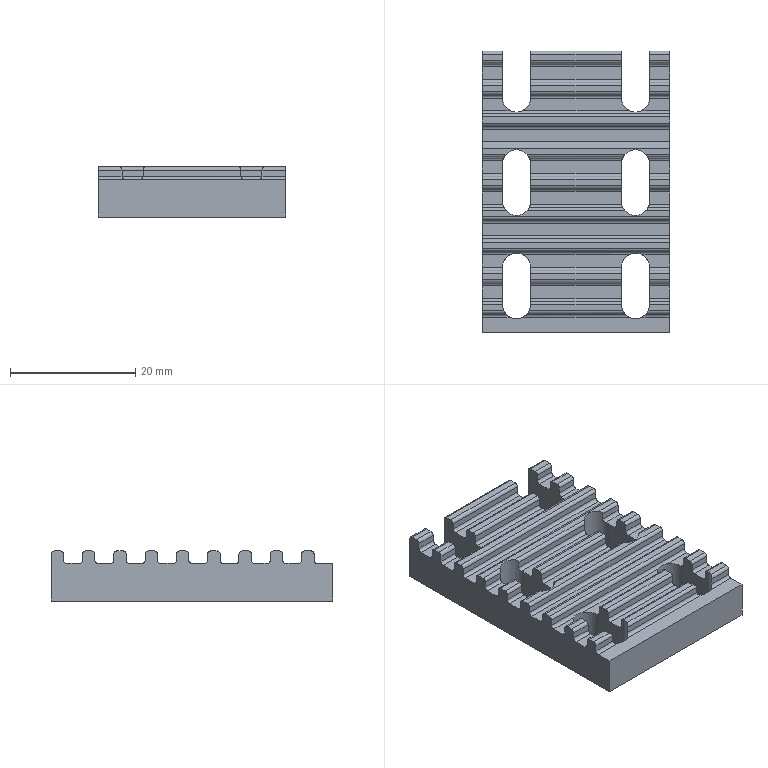Component | SolidWorks | 01000000A08017AAdjustingBeltPressureBlock(Battery)122-1 | 1 solid | 195 faces | box 30 x 45 x 8 mm | volume 7442 mm3 | plane 98 | cylinder 97 | commonest cylinder face diameters 1 x81 4.5 x16
build123d program:
from build123d import *

# Parameters (mm, degrees)
BOSS_EXTRUDE1_DEPTH            = 15
FILLET1_R                      = 0.5
F_4_5_4_5_DIAMETER_HOLE1_D     = 4.5
F_4_5_4_5_DIAMETER_HOLE1_DEPTH = 10
F_4_5_4_5_DIAMETER_HOLE1_TIP   = 1.352
SKETCH8_W                      = 3
SKETCH8_H                      = 30
CUT_EXTRUDE2_DEPTH             = 48.812
CUT_EXTRUDE1_DEPTH             = 46.31


with BuildPart() as part:
    # Sketch1 → Boss-Extrude1 (new, symmetric)
    with BuildSketch(Plane.XY):
        Polygon((27, 0), (27, 2), (30, 2), (30, 0), (32, 0), (32, 2), (35, 2), (35, 0), (37, 0), (37, 2), (40, 2), (40, 0), (42, 0), (42, 2), (45, 2), (45, 8), (-3, 8), (-3, 2), (0, 2), (0, 0), (2, 0), (2, 2), (5, 2), (5, 0), (7, 0), (7, 2), (10, 2), (10, 0), (12, 0), (12, 2), (15, 2), (15, 0), (17, 0), (17, 2), (20, 2), (20, 0), (22, 0), (22, 2), (25, 2), (25, 0), align=None)
    extrude(amount=BOSS_EXTRUDE1_DEPTH, both=True)

    # Fillet1
    fillet1_edges = [part.edges().sort_by_distance(p)[0] for p in [
        (35, 2, 0),
        (32, 2, 0),
        (32, 0, 0),
        (30, 0, 0),
        (30, 2, 0),
        (27, 2, 0),
        (27, 0, 0),
        (25, 0, 0),
        (25, 2, 0),
        (22, 2, 0),
        (22, 0, 0),
        (20, 0, 0),
        (20, 2, 0),
        (17, 2, 0),
        (17, 0, 0),
        (15, 0, 0),
        (15, 2, 0),
        (12, 2, 0),
        (12, 0, 0),
        (10, 0, 0),
        (10, 2, 0),
        (7, 2, 0),
        (7, 0, 0),
        (5, 0, 0),
        (5, 2, 0),
        (2, 2, 0),
        (2, 0, 0),
        (0, 0, 0),
        (0, 2, 0),
        (42, 0, 0),
        (40, 0, 0),
        (40, 2, 0),
        (37, 2, 0),
        (37, 0, 0),
        (35, 0, 0),
    ]]
    fillet(fillet1_edges, radius=FILLET1_R)

    # 4.5 _4.5_ Diameter Hole1
    with Locations(Plane(origin=(0, 8, 0), x_dir=(-1, 0, 0), z_dir=(0, 1, 0))):
        with Locations((-4.5, -9.5), (-37.5, -9.5), (-4.5, 9.5), (-37.5, 9.5), (-21, 9.5), (-21, -9.5)):
            Hole(F_4_5_4_5_DIAMETER_HOLE1_D / 2, depth=F_4_5_4_5_DIAMETER_HOLE1_DEPTH)
            with Locations((0, 0, -(F_4_5_4_5_DIAMETER_HOLE1_DEPTH + F_4_5_4_5_DIAMETER_HOLE1_TIP / 2))):  # 118° drill point
                Cone(0, F_4_5_4_5_DIAMETER_HOLE1_D / 2, F_4_5_4_5_DIAMETER_HOLE1_TIP, mode=Mode.SUBTRACT)

    # Sketch8 → Cut-Extrude2 (cut, through all)
    with BuildSketch(Plane.XZ.offset(-2)):
        with Locations((43.5, 0)):
            Rectangle(SKETCH8_W, SKETCH8_H)
    extrude(amount=-CUT_EXTRUDE2_DEPTH, mode=Mode.SUBTRACT)

    # Sketch5 → Cut-Extrude1 (cut, through all)
    with BuildSketch(Plane(origin=(0, 8, 0), x_dir=(1, 0, 0), z_dir=(0, 1, 0))):
        with BuildLine():
            Line((34.5, 7.25), (42, 7.25))
            Line((42, 7.25), (42, 11.75))
            Line((42, 11.75), (34.5, 11.75))
            ThreePointArc((34.5, 11.75), (32.25, 9.5), (34.5, 7.25))
        make_face()
        with BuildLine():
            Line((42, -11.75), (42, -7.25))
            Line((42, -7.25), (34.5, -7.25))
            ThreePointArc((34.5, -7.25), (32.25, -9.5), (34.5, -11.75))
            Line((34.5, -11.75), (42, -11.75))
        make_face()
        with BuildLine():
            Line((7.5, 7.25), (1.5, 7.25))
            ThreePointArc((1.5, 7.25), (-0.75, 9.5), (1.5, 11.75))
            Line((1.5, 11.75), (7.5, 11.75))
            ThreePointArc((7.5, 11.75), (9.75, 9.5), (7.5, 7.25))
        make_face()
        with BuildLine():
            Line((7.5, -11.75), (1.5, -11.75))
            ThreePointArc((1.5, -11.75), (-0.75, -9.5), (1.5, -7.25))
            Line((1.5, -7.25), (7.5, -7.25))
            ThreePointArc((7.5, -7.25), (9.75, -9.5), (7.5, -11.75))
        make_face()
        with BuildLine():
            Line((18, 11.75), (24, 11.75))
            ThreePointArc((24, 11.75), (26.25, 9.5), (24, 7.25))
            Line((24, 7.25), (18, 7.25))
            ThreePointArc((18, 7.25), (15.75, 9.5), (18, 11.75))
        make_face()
        with BuildLine():
            Line((18, -7.25), (24, -7.25))
            ThreePointArc((24, -7.25), (26.25, -9.5), (24, -11.75))
            Line((24, -11.75), (18, -11.75))
            ThreePointArc((18, -11.75), (15.75, -9.5), (18, -7.25))
        make_face()
    extrude(amount=-CUT_EXTRUDE1_DEPTH, mode=Mode.SUBTRACT)


solid = part.part

# Placed as in the assembly
solid = solid.moved(Location((-212.479, -46.348, 874.07), (-90, -90, 0)))